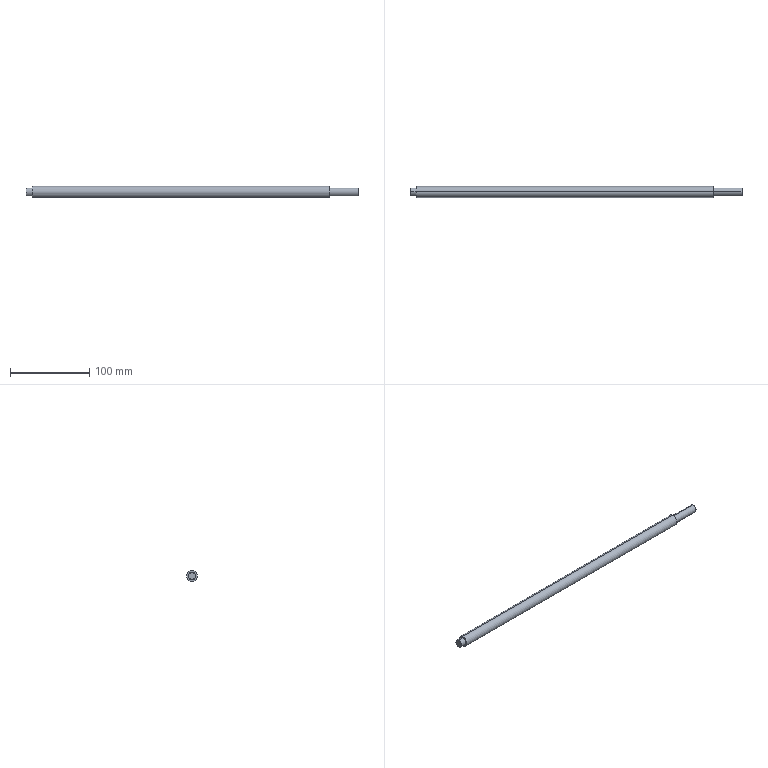Component | SolidWorks | CS021-T-BallScrew16x4(ZYCS002)-1 | 1 solid | 12 faces | box 419 x 14 x 14 mm | volume 61177 mm3 | cylinder 6 | plane 4 | cone 2 | commonest cylinder face diameters 10 x4 14 x2 | material 45
build123d program:
from build123d import *

# Parameters (mm, degrees)
SKETCH1_R           = 7
BOSS_EXTRUDE1_DEPTH = 187.5
SKETCH2_R           = 5
BOSS_EXTRUDE2_DEPTH = 8
CHAMFER1_SIZE       = 0.6
BOSS_EXTRUDE3_START = 36
SKETCH4_R           = 5
BOSS_EXTRUDE3_DEPTH = 36


with BuildPart() as part:
    # Sketch1 → Boss-Extrude1 (new, symmetric)
    with BuildSketch(Plane(origin=(0, 0, 0), x_dir=(0, 0, -1), z_dir=(1, 0, 0))):
        Circle(SKETCH1_R)
    extrude(amount=BOSS_EXTRUDE1_DEPTH, both=True)

    # Sketch2 → Boss-Extrude2 (add)
    with BuildSketch(Plane.ZY.offset(187.5)):
        with Locations(Location((0, 0, 0), (0, 0, 180))):
            Circle(SKETCH2_R)
    extrude(amount=BOSS_EXTRUDE2_DEPTH)

    # Chamfer1
    chamfer1_edges = [part.edges().sort_by_distance(p)[0] for p in [
        (-195.5, 0, 5),
    ]]
    chamfer(chamfer1_edges, length=CHAMFER1_SIZE)

    # Sketch4 → Boss-Extrude3 (add)
    with BuildSketch(Plane(origin=(187.5, 0, 0), x_dir=(0, 0, -1), z_dir=(1, 0, 0)).offset(BOSS_EXTRUDE3_START)):
        Circle(SKETCH4_R)
    extrude(amount=-BOSS_EXTRUDE3_DEPTH)


solid = part.part

# Placed as in the assembly
solid = solid.moved(Location((33.449, 84.817, 0), (0, 0, 0)))
STEP:
#1=COLOUR_RGB('',0.7922,0.8196,0.9333);
#2=FILL_AREA_STYLE_COLOUR('',#1);
#3=FILL_AREA_STYLE('',(#2));
#4=SURFACE_STYLE_FILL_AREA(#3);
#5=SURFACE_SIDE_STYLE('',(#4));
#6=SURFACE_STYLE_USAGE(.BOTH.,#5);
#7=PRESENTATION_STYLE_ASSIGNMENT((#6));
#8=CARTESIAN_POINT('',(10.116,3.362,0.1955));
#9=VERTEX_POINT('',#8);
#10=CARTESIAN_POINT('',(10.116,3.316,-0.1955));
#11=VERTEX_POINT('',#10);
#12=CARTESIAN_POINT('',(10.116,3.339,-0.));
#13=DIRECTION('',(1.,-0.,-0.));
#14=DIRECTION('',(0.,0.118,0.993));
#15=AXIS2_PLACEMENT_3D('',#12,#13,#14);
#16=CIRCLE('',#15,0.1969);
#17=EDGE_CURVE('',#9,#11,#16,.T.);
#18=ORIENTED_EDGE('',*,*,#17,.F.);
#19=CARTESIAN_POINT('',(8.699,3.362,0.1955));
#20=VERTEX_POINT('',#19);
#21=CARTESIAN_POINT('',(10.116,3.362,0.1955));
#22=DIRECTION('',(-1.,0.,0.));
#23=VECTOR('',#22,39.37);
#24=LINE('',#21,#23);
#25=EDGE_CURVE('',#9,#20,#24,.T.);
#26=ORIENTED_EDGE('',*,*,#25,.T.);
#27=CARTESIAN_POINT('',(8.699,3.316,-0.1955));
#28=VERTEX_POINT('',#27);
#29=CARTESIAN_POINT('',(8.699,3.339,-0.));
#30=DIRECTION('',(1.,-0.,-0.));
#31=DIRECTION('',(0.,0.118,0.993));
#32=AXIS2_PLACEMENT_3D('',#29,#30,#31);
#33=CIRCLE('',#32,0.1969);
#34=EDGE_CURVE('',#20,#28,#33,.T.);
#35=ORIENTED_EDGE('',*,*,#34,.T.);
#36=CARTESIAN_POINT('',(10.116,3.316,-0.1955));
#37=DIRECTION('',(-1.,0.,0.));
#38=VECTOR('',#37,39.37);
#39=LINE('',#36,#38);
#40=EDGE_CURVE('',#11,#28,#39,.T.);
#41=ORIENTED_EDGE('',*,*,#40,.F.);
#42=EDGE_LOOP('',(#18,#26,#35,#41));
#43=FACE_OUTER_BOUND('',#42,.T.);
#44=CARTESIAN_POINT('',(10.116,3.339,-0.));
#45=DIRECTION('',(-1.,0.,0.));
#46=DIRECTION('',(0.,-0.118,-0.993));
#47=AXIS2_PLACEMENT_3D('',#44,#45,#46);
#48=CYLINDRICAL_SURFACE('',#47,0.1969);
#49=ADVANCED_FACE('',(#43),#48,.T.);
#50=CARTESIAN_POINT('',(-6.38,3.319,-0.172));
#51=VERTEX_POINT('',#50);
#52=CARTESIAN_POINT('',(-6.38,3.36,0.172));
#53=VERTEX_POINT('',#52);
#54=CARTESIAN_POINT('',(-6.38,3.339,0.));
#55=DIRECTION('',(-1.,0.,0.));
#56=DIRECTION('',(0.,-0.118,-0.993));
#57=AXIS2_PLACEMENT_3D('',#54,#55,#56);
#58=CIRCLE('',#57,0.1732);
#59=EDGE_CURVE('',#51,#53,#58,.T.);
#60=ORIENTED_EDGE('',*,*,#59,.F.);
#61=CARTESIAN_POINT('',(-6.356,3.316,-0.1955));
#62=VERTEX_POINT('',#61);
#63=CARTESIAN_POINT('',(-6.38,3.319,-0.172));
#64=DIRECTION('',(0.7071,-0.08343,-0.7022));
#65=VECTOR('',#64,39.37);
#66=LINE('',#63,#65);
#67=EDGE_CURVE('',#51,#62,#66,.T.);
#68=ORIENTED_EDGE('',*,*,#67,.T.);
#69=CARTESIAN_POINT('',(-6.356,3.362,0.1955));
#70=VERTEX_POINT('',#69);
#71=CARTESIAN_POINT('',(-6.356,3.339,0.));
#72=DIRECTION('',(1.,-0.,-0.));
#73=DIRECTION('',(0.,-0.118,-0.993));
#74=AXIS2_PLACEMENT_3D('',#71,#72,#73);
#75=CIRCLE('',#74,0.1969);
#76=EDGE_CURVE('',#70,#62,#75,.T.);
#77=ORIENTED_EDGE('',*,*,#76,.F.);
#78=CARTESIAN_POINT('',(-6.38,3.36,0.172));
#79=DIRECTION('',(0.7071,0.08343,0.7022));
#80=VECTOR('',#79,39.37);
#81=LINE('',#78,#80);
#82=EDGE_CURVE('',#53,#70,#81,.T.);
#83=ORIENTED_EDGE('',*,*,#82,.F.);
#84=EDGE_LOOP('',(#60,#68,#77,#83));
#85=FACE_OUTER_BOUND('',#84,.T.);
#86=CARTESIAN_POINT('',(-6.38,3.339,0.));
#87=DIRECTION('',(1.,-0.,-0.));
#88=DIRECTION('',(0.,0.118,0.993));
#89=AXIS2_PLACEMENT_3D('',#86,#87,#88);
#90=CONICAL_SURFACE('',#89,0.1732,0.7854);
#91=ADVANCED_FACE('',(#85),#90,.T.);
#92=ORIENTED_EDGE('',*,*,#76,.T.);
#93=CARTESIAN_POINT('',(-6.065,3.316,-0.1955));
#94=VERTEX_POINT('',#93);
#95=CARTESIAN_POINT('',(-6.38,3.316,-0.1955));
#96=DIRECTION('',(1.,-0.,-0.));
#97=VECTOR('',#96,39.37);
#98=LINE('',#95,#97);
#99=EDGE_CURVE('',#62,#94,#98,.T.);
#100=ORIENTED_EDGE('',*,*,#99,.T.);
#101=CARTESIAN_POINT('',(-6.065,3.362,0.1955));
#102=VERTEX_POINT('',#101);
#103=CARTESIAN_POINT('',(-6.065,3.339,-0.));
#104=DIRECTION('',(-1.,0.,0.));
#105=DIRECTION('',(0.,0.118,0.993));
#106=AXIS2_PLACEMENT_3D('',#103,#104,#105);
#107=CIRCLE('',#106,0.1969);
#108=EDGE_CURVE('',#94,#102,#107,.T.);
#109=ORIENTED_EDGE('',*,*,#108,.T.);
#110=CARTESIAN_POINT('',(-6.38,3.362,0.1955));
#111=DIRECTION('',(1.,-0.,-0.));
#112=VECTOR('',#111,39.37);
#113=LINE('',#110,#112);
#114=EDGE_CURVE('',#70,#102,#113,.T.);
#115=ORIENTED_EDGE('',*,*,#114,.F.);
#116=EDGE_LOOP('',(#92,#100,#109,#115));
#117=FACE_OUTER_BOUND('',#116,.T.);
#118=CARTESIAN_POINT('',(-6.38,3.339,0.));
#119=DIRECTION('',(1.,-0.,-0.));
#120=DIRECTION('',(0.,0.118,0.993));
#121=AXIS2_PLACEMENT_3D('',#118,#119,#120);
#122=CYLINDRICAL_SURFACE('',#121,0.1969);
#123=ADVANCED_FACE('',(#117),#122,.T.);
#124=CARTESIAN_POINT('',(8.699,3.372,0.2737));
#125=VERTEX_POINT('',#124);
#126=CARTESIAN_POINT('',(8.699,3.307,-0.2737));
#127=VERTEX_POINT('',#126);
#128=CARTESIAN_POINT('',(8.699,3.339,-0.));
#129=DIRECTION('',(1.,-0.,-0.));
#130=DIRECTION('',(0.,0.118,0.993));
#131=AXIS2_PLACEMENT_3D('',#128,#129,#130);
#132=CIRCLE('',#131,0.2756);
#133=EDGE_CURVE('',#125,#127,#132,.T.);
#134=ORIENTED_EDGE('',*,*,#133,.F.);
#135=CARTESIAN_POINT('',(-6.065,3.372,0.2737));
#136=VERTEX_POINT('',#135);
#137=CARTESIAN_POINT('',(8.699,3.372,0.2737));
#138=DIRECTION('',(-1.,0.,0.));
#139=VECTOR('',#138,39.37);
#140=LINE('',#137,#139);
#141=EDGE_CURVE('',#125,#136,#140,.T.);
#142=ORIENTED_EDGE('',*,*,#141,.T.);
#143=CARTESIAN_POINT('',(-6.065,3.307,-0.2737));
#144=VERTEX_POINT('',#143);
#145=CARTESIAN_POINT('',(-6.065,3.339,-0.));
#146=DIRECTION('',(1.,-0.,-0.));
#147=DIRECTION('',(0.,0.118,0.993));
#148=AXIS2_PLACEMENT_3D('',#145,#146,#147);
#149=CIRCLE('',#148,0.2756);
#150=EDGE_CURVE('',#136,#144,#149,.T.);
#151=ORIENTED_EDGE('',*,*,#150,.T.);
#152=CARTESIAN_POINT('',(8.699,3.307,-0.2737));
#153=DIRECTION('',(-1.,0.,0.));
#154=VECTOR('',#153,39.37);
#155=LINE('',#152,#154);
#156=EDGE_CURVE('',#127,#144,#155,.T.);
#157=ORIENTED_EDGE('',*,*,#156,.F.);
#158=EDGE_LOOP('',(#134,#142,#151,#157));
#159=FACE_OUTER_BOUND('',#158,.T.);
#160=CARTESIAN_POINT('',(8.699,3.339,-0.));
#161=DIRECTION('',(-1.,0.,0.));
#162=DIRECTION('',(0.,-0.118,-0.993));
#163=AXIS2_PLACEMENT_3D('',#160,#161,#162);
#164=CYLINDRICAL_SURFACE('',#163,0.2756);
#165=ADVANCED_FACE('',(#159),#164,.T.);
#166=CARTESIAN_POINT('',(8.699,3.339,-0.));
#167=DIRECTION('',(1.,-0.,-0.));
#168=DIRECTION('',(0.,0.118,0.993));
#169=AXIS2_PLACEMENT_3D('',#166,#167,#168);
#170=CIRCLE('',#169,0.2756);
#171=EDGE_CURVE('',#127,#125,#170,.T.);
#172=ORIENTED_EDGE('',*,*,#171,.T.);
#173=ORIENTED_EDGE('',*,*,#133,.T.);
#174=EDGE_LOOP('',(#172,#173));
#175=FACE_OUTER_BOUND('',#174,.T.);
#176=CARTESIAN_POINT('',(8.699,3.339,-0.));
#177=DIRECTION('',(1.,-0.,-0.));
#178=DIRECTION('',(0.,0.118,0.993));
#179=AXIS2_PLACEMENT_3D('',#176,#177,#178);
#180=CIRCLE('',#179,0.1969);
#181=EDGE_CURVE('',#28,#20,#180,.T.);
#182=ORIENTED_EDGE('',*,*,#181,.F.);
#183=ORIENTED_EDGE('',*,*,#34,.F.);
#184=EDGE_LOOP('',(#182,#183));
#185=FACE_BOUND('',#184,.T.);
#186=CARTESIAN_POINT('',(8.699,3.339,-0.));
#187=DIRECTION('',(1.,-0.,-0.));
#188=DIRECTION('',(0.,0.118,0.993));
#189=AXIS2_PLACEMENT_3D('',#186,#187,#188);
#190=PLANE('',#189);
#191=ADVANCED_FACE('',(#175,#185),#190,.T.);
#192=CARTESIAN_POINT('',(-6.065,3.339,-0.));
#193=DIRECTION('',(1.,-0.,-0.));
#194=DIRECTION('',(0.,0.118,0.993));
#195=AXIS2_PLACEMENT_3D('',#192,#193,#194);
#196=CIRCLE('',#195,0.2756);
#197=EDGE_CURVE('',#144,#136,#196,.T.);
#198=ORIENTED_EDGE('',*,*,#197,.F.);
#199=ORIENTED_EDGE('',*,*,#150,.F.);
#200=EDGE_LOOP('',(#198,#199));
#201=FACE_OUTER_BOUND('',#200,.T.);
#202=CARTESIAN_POINT('',(-6.065,3.339,-0.));
#203=DIRECTION('',(-1.,0.,0.));
#204=DIRECTION('',(0.,0.118,0.993));
#205=AXIS2_PLACEMENT_3D('',#202,#203,#204);
#206=CIRCLE('',#205,0.1969);
#207=EDGE_CURVE('',#102,#94,#206,.T.);
#208=ORIENTED_EDGE('',*,*,#207,.F.);
#209=ORIENTED_EDGE('',*,*,#108,.F.);
#210=EDGE_LOOP('',(#208,#209));
#211=FACE_BOUND('',#210,.T.);
#212=CARTESIAN_POINT('',(-6.065,3.339,-0.));
#213=DIRECTION('',(1.,-0.,-0.));
#214=DIRECTION('',(0.,0.118,0.993));
#215=AXIS2_PLACEMENT_3D('',#212,#213,#214);
#216=PLANE('',#215);
#217=ADVANCED_FACE('',(#201,#211),#216,.F.);
#218=ORIENTED_EDGE('',*,*,#141,.F.);
#219=ORIENTED_EDGE('',*,*,#171,.F.);
#220=ORIENTED_EDGE('',*,*,#156,.T.);
#221=ORIENTED_EDGE('',*,*,#197,.T.);
#222=EDGE_LOOP('',(#218,#219,#220,#221));
#223=FACE_OUTER_BOUND('',#222,.T.);
#224=CARTESIAN_POINT('',(8.699,3.339,-0.));
#225=DIRECTION('',(-1.,0.,0.));
#226=DIRECTION('',(0.,-0.118,-0.993));
#227=AXIS2_PLACEMENT_3D('',#224,#225,#226);
#228=CYLINDRICAL_SURFACE('',#227,0.2756);
#229=ADVANCED_FACE('',(#223),#228,.T.);
#230=ORIENTED_EDGE('',*,*,#99,.F.);
#231=CARTESIAN_POINT('',(-6.356,3.339,0.));
#232=DIRECTION('',(1.,-0.,-0.));
#233=DIRECTION('',(0.,-0.118,-0.993));
#234=AXIS2_PLACEMENT_3D('',#231,#232,#233);
#235=CIRCLE('',#234,0.1969);
#236=EDGE_CURVE('',#62,#70,#235,.T.);
#237=ORIENTED_EDGE('',*,*,#236,.T.);
#238=ORIENTED_EDGE('',*,*,#114,.T.);
#239=ORIENTED_EDGE('',*,*,#207,.T.);
#240=EDGE_LOOP('',(#230,#237,#238,#239));
#241=FACE_OUTER_BOUND('',#240,.T.);
#242=CARTESIAN_POINT('',(-6.38,3.339,0.));
#243=DIRECTION('',(1.,-0.,-0.));
#244=DIRECTION('',(0.,0.118,0.993));
#245=AXIS2_PLACEMENT_3D('',#242,#243,#244);
#246=CYLINDRICAL_SURFACE('',#245,0.1969);
#247=ADVANCED_FACE('',(#241),#246,.T.);
#248=CARTESIAN_POINT('',(-6.38,3.339,0.));
#249=DIRECTION('',(-1.,0.,0.));
#250=DIRECTION('',(0.,-0.118,-0.993));
#251=AXIS2_PLACEMENT_3D('',#248,#249,#250);
#252=CIRCLE('',#251,0.1732);
#253=EDGE_CURVE('',#53,#51,#252,.T.);
#254=ORIENTED_EDGE('',*,*,#253,.T.);
#255=ORIENTED_EDGE('',*,*,#59,.T.);
#256=EDGE_LOOP('',(#254,#255));
#257=FACE_OUTER_BOUND('',#256,.T.);
#258=CARTESIAN_POINT('',(-6.38,3.339,0.));
#259=DIRECTION('',(-1.,0.,0.));
#260=DIRECTION('',(-0.,-0.118,-0.993));
#261=AXIS2_PLACEMENT_3D('',#258,#259,#260);
#262=PLANE('',#261);
#263=ADVANCED_FACE('',(#257),#262,.T.);
#264=ORIENTED_EDGE('',*,*,#67,.F.);
#265=ORIENTED_EDGE('',*,*,#253,.F.);
#266=ORIENTED_EDGE('',*,*,#82,.T.);
#267=ORIENTED_EDGE('',*,*,#236,.F.);
#268=EDGE_LOOP('',(#264,#265,#266,#267));
#269=FACE_OUTER_BOUND('',#268,.T.);
#270=CARTESIAN_POINT('',(-6.38,3.339,0.));
#271=DIRECTION('',(1.,-0.,-0.));
#272=DIRECTION('',(0.,0.118,0.993));
#273=AXIS2_PLACEMENT_3D('',#270,#271,#272);
#274=CONICAL_SURFACE('',#273,0.1732,0.7854);
#275=ADVANCED_FACE('',(#269),#274,.T.);
#276=ORIENTED_EDGE('',*,*,#25,.F.);
#277=CARTESIAN_POINT('',(10.116,3.339,-0.));
#278=DIRECTION('',(1.,-0.,-0.));
#279=DIRECTION('',(0.,0.118,0.993));
#280=AXIS2_PLACEMENT_3D('',#277,#278,#279);
#281=CIRCLE('',#280,0.1969);
#282=EDGE_CURVE('',#11,#9,#281,.T.);
#283=ORIENTED_EDGE('',*,*,#282,.F.);
#284=ORIENTED_EDGE('',*,*,#40,.T.);
#285=ORIENTED_EDGE('',*,*,#181,.T.);
#286=EDGE_LOOP('',(#276,#283,#284,#285));
#287=FACE_OUTER_BOUND('',#286,.T.);
#288=CARTESIAN_POINT('',(10.116,3.339,-0.));
#289=DIRECTION('',(-1.,0.,0.));
#290=DIRECTION('',(0.,-0.118,-0.993));
#291=AXIS2_PLACEMENT_3D('',#288,#289,#290);
#292=CYLINDRICAL_SURFACE('',#291,0.1969);
#293=ADVANCED_FACE('',(#287),#292,.T.);
#294=ORIENTED_EDGE('',*,*,#282,.T.);
#295=ORIENTED_EDGE('',*,*,#17,.T.);
#296=EDGE_LOOP('',(#294,#295));
#297=FACE_OUTER_BOUND('',#296,.T.);
#298=CARTESIAN_POINT('',(10.116,3.339,-0.));
#299=DIRECTION('',(1.,-0.,-0.));
#300=DIRECTION('',(0.,0.118,0.993));
#301=AXIS2_PLACEMENT_3D('',#298,#299,#300);
#302=PLANE('',#301);
#303=ADVANCED_FACE('',(#297),#302,.T.);
#304=CLOSED_SHELL('',(#49,#91,#123,#165,#191,#217,#229,#247,#263,#275,#293,#303));
#305=MANIFOLD_SOLID_BREP('',#304);
#306=STYLED_ITEM('',(#7),#305);
#307=PRESENTATION_LAYER_ASSIGNMENT('','',(#306));
#308=CARTESIAN_POINT('',(0.,0.,0.));
#309=DIRECTION('',(0.,0.,1.));
#310=DIRECTION('',(1.,0.,0.));
#311=AXIS2_PLACEMENT_3D('',#308,#309,#310);
#312=(LENGTH_UNIT()NAMED_UNIT(*)SI_UNIT($,.METRE.));
#313=LENGTH_MEASURE_WITH_UNIT(LENGTH_MEASURE(0.0254),#312);
#314=DIMENSIONAL_EXPONENTS(1.,0.,0.,0.,0.,0.,0.);
#315=(CONVERSION_BASED_UNIT('',#313)LENGTH_UNIT()NAMED_UNIT(#314));
#316=UNCERTAINTY_MEASURE_WITH_UNIT(LENGTH_MEASURE(0.00001),#315,'','');
#317=(NAMED_UNIT(*)PLANE_ANGLE_UNIT()SI_UNIT($,.RADIAN.));
#318=(NAMED_UNIT(*)SI_UNIT($,.STERADIAN.)SOLID_ANGLE_UNIT());
#319=(GEOMETRIC_REPRESENTATION_CONTEXT(3)GLOBAL_UNCERTAINTY_ASSIGNED_CONTEXT((#316))GLOBAL_UNIT_ASSIGNED_CONTEXT((#315,#317,#318))REPRESENTATION_CONTEXT('',''));
#320=ADVANCED_BREP_SHAPE_REPRESENTATION('',(#305,#311),#319);
#321=(LENGTH_UNIT()NAMED_UNIT(*)SI_UNIT($,.METRE.));
#322=LENGTH_MEASURE_WITH_UNIT(LENGTH_MEASURE(0.0254),#321);
#323=DIMENSIONAL_EXPONENTS(1.,0.,0.,0.,0.,0.,0.);
#324=(CONVERSION_BASED_UNIT('',#322)LENGTH_UNIT()NAMED_UNIT(#323));
#325=UNCERTAINTY_MEASURE_WITH_UNIT(LENGTH_MEASURE(0.00001),#324,'','');
#326=(NAMED_UNIT(*)PLANE_ANGLE_UNIT()SI_UNIT($,.RADIAN.));
#327=(NAMED_UNIT(*)SI_UNIT($,.STERADIAN.)SOLID_ANGLE_UNIT());
#328=(GEOMETRIC_REPRESENTATION_CONTEXT(3)GLOBAL_UNCERTAINTY_ASSIGNED_CONTEXT((#325))GLOBAL_UNIT_ASSIGNED_CONTEXT((#324,#326,#327))REPRESENTATION_CONTEXT('',''));
#329=MECHANICAL_DESIGN_GEOMETRIC_PRESENTATION_REPRESENTATION('',(#306),#328);